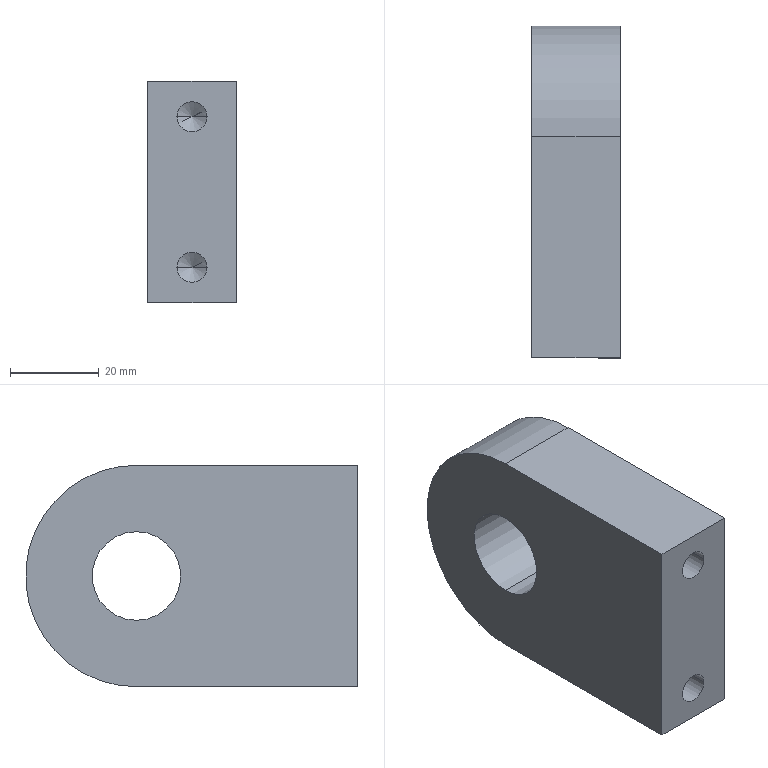Component | SolidWorks | BracketOne-1 | 1 solid | 16 faces | box 20 x 75 x 50 mm | volume 62431 mm3 | cylinder 7 | plane 5 | cone 4 | commonest cylinder face diameters 6.8 x4 20 x2 50 x1
build123d program:
from build123d import *

# Parameters (mm, degrees)
SKETCH1_R             = 10
BOSS_EXTRUDE1_DEPTH   = 20
M8_TAPPED_HOLE1_D     = 6.8
M8_TAPPED_HOLE1_DEPTH = 12
M8_TAPPED_HOLE1_TIP   = 2.043


with BuildPart() as part:
    # Sketch1 → Boss-Extrude1 (new body)
    with BuildSketch(Plane.XY):
        with BuildLine():
            Line((-25, 25), (-25, -25))
            Line((-25, -25), (25, -25))
            Line((25, -25), (25, 25))
            ThreePointArc((25, 25), (0, 50), (-25, 25))
        make_face()
        with Locations((0, 25)):
            Circle(SKETCH1_R, mode=Mode.SUBTRACT)
    extrude(amount=BOSS_EXTRUDE1_DEPTH)

    # M8 Tapped Hole1
    with Locations(Plane(origin=(0, -25, 0), x_dir=(-1, 0, 0), z_dir=(0, -1, 0))):
        with Locations((17, -10), (-17, -10)):
            Hole(M8_TAPPED_HOLE1_D / 2, depth=M8_TAPPED_HOLE1_DEPTH)
            with Locations((0, 0, -(M8_TAPPED_HOLE1_DEPTH + M8_TAPPED_HOLE1_TIP / 2))):  # 118° drill point
                Cone(0, M8_TAPPED_HOLE1_D / 2, M8_TAPPED_HOLE1_TIP, mode=Mode.SUBTRACT)


solid = part.part

# Placed as in the assembly
solid = solid.moved(Location((70.246, 37, 355.671), (0, 90, 0)))
STEP:
#1=COLOUR_RGB('',0.7922,0.8196,0.9333);
#2=FILL_AREA_STYLE_COLOUR('',#1);
#3=FILL_AREA_STYLE('',(#2));
#4=SURFACE_STYLE_FILL_AREA(#3);
#5=SURFACE_SIDE_STYLE('',(#4));
#6=SURFACE_STYLE_USAGE(.BOTH.,#5);
#7=PRESENTATION_STYLE_ASSIGNMENT((#6));
#8=CARTESIAN_POINT('',(3.293,0.9449,14.672));
#9=VERTEX_POINT('',#8);
#10=CARTESIAN_POINT('',(3.025,0.9449,14.672));
#11=VERTEX_POINT('',#10);
#12=CARTESIAN_POINT('',(3.159,0.9449,14.672));
#13=DIRECTION('',(0.,-1.,-0.));
#14=DIRECTION('',(-1.,0.,0.));
#15=AXIS2_PLACEMENT_3D('',#12,#13,#14);
#16=CIRCLE('',#15,0.1339);
#17=EDGE_CURVE('',#9,#11,#16,.T.);
#18=ORIENTED_EDGE('',*,*,#17,.F.);
#19=CARTESIAN_POINT('',(3.293,0.4724,14.672));
#20=VERTEX_POINT('',#19);
#21=CARTESIAN_POINT('',(3.293,0.4724,14.672));
#22=DIRECTION('',(0.,-1.,-0.));
#23=VECTOR('',#22,39.37);
#24=LINE('',#21,#23);
#25=EDGE_CURVE('',#9,#20,#24,.T.);
#26=ORIENTED_EDGE('',*,*,#25,.T.);
#27=CARTESIAN_POINT('',(3.025,0.4724,14.672));
#28=VERTEX_POINT('',#27);
#29=CARTESIAN_POINT('',(3.159,0.4724,14.672));
#30=DIRECTION('',(0.,-1.,-0.));
#31=DIRECTION('',(-1.,0.,0.));
#32=AXIS2_PLACEMENT_3D('',#29,#30,#31);
#33=CIRCLE('',#32,0.1339);
#34=EDGE_CURVE('',#20,#28,#33,.T.);
#35=ORIENTED_EDGE('',*,*,#34,.T.);
#36=CARTESIAN_POINT('',(3.025,0.4724,14.672));
#37=DIRECTION('',(0.,-1.,-0.));
#38=VECTOR('',#37,39.37);
#39=LINE('',#36,#38);
#40=EDGE_CURVE('',#11,#28,#39,.T.);
#41=ORIENTED_EDGE('',*,*,#40,.F.);
#42=EDGE_LOOP('',(#18,#26,#35,#41));
#43=FACE_OUTER_BOUND('',#42,.T.);
#44=CARTESIAN_POINT('',(3.159,0.4724,14.672));
#45=DIRECTION('',(0.,-1.,-0.));
#46=DIRECTION('',(-1.,0.,0.));
#47=AXIS2_PLACEMENT_3D('',#44,#45,#46);
#48=CYLINDRICAL_SURFACE('',#47,0.1339);
#49=ADVANCED_FACE('',(#43),#48,.F.);
#50=CARTESIAN_POINT('',(3.159,1.025,14.672));
#51=VERTEX_POINT('',#50);
#52=CARTESIAN_POINT('',(3.025,0.9449,14.672));
#53=DIRECTION('',(-0.8572,-0.515,0.));
#54=VECTOR('',#53,39.37);
#55=LINE('',#52,#54);
#56=EDGE_CURVE('',#51,#11,#55,.T.);
#57=ORIENTED_EDGE('',*,*,#56,.F.);
#58=CARTESIAN_POINT('',(3.293,0.9449,14.672));
#59=DIRECTION('',(0.8572,-0.515,-0.));
#60=VECTOR('',#59,39.37);
#61=LINE('',#58,#60);
#62=EDGE_CURVE('',#51,#9,#61,.T.);
#63=ORIENTED_EDGE('',*,*,#62,.T.);
#64=ORIENTED_EDGE('',*,*,#17,.T.);
#65=EDGE_LOOP('',(#57,#63,#64));
#66=FACE_OUTER_BOUND('',#65,.T.);
#67=CARTESIAN_POINT('',(3.159,0.9449,14.672));
#68=DIRECTION('',(0.,-1.,-0.));
#69=DIRECTION('',(-1.,0.,0.));
#70=AXIS2_PLACEMENT_3D('',#67,#68,#69);
#71=CONICAL_SURFACE('',#70,0.1339,1.03);
#72=ADVANCED_FACE('',(#66),#71,.F.);
#73=CARTESIAN_POINT('',(3.293,0.9449,13.334));
#74=VERTEX_POINT('',#73);
#75=CARTESIAN_POINT('',(3.025,0.9449,13.334));
#76=VERTEX_POINT('',#75);
#77=CARTESIAN_POINT('',(3.159,0.9449,13.334));
#78=DIRECTION('',(0.,-1.,-0.));
#79=DIRECTION('',(-1.,0.,0.));
#80=AXIS2_PLACEMENT_3D('',#77,#78,#79);
#81=CIRCLE('',#80,0.1339);
#82=EDGE_CURVE('',#74,#76,#81,.T.);
#83=ORIENTED_EDGE('',*,*,#82,.F.);
#84=CARTESIAN_POINT('',(3.293,0.4724,13.334));
#85=VERTEX_POINT('',#84);
#86=CARTESIAN_POINT('',(3.293,0.4724,13.334));
#87=DIRECTION('',(0.,-1.,-0.));
#88=VECTOR('',#87,39.37);
#89=LINE('',#86,#88);
#90=EDGE_CURVE('',#74,#85,#89,.T.);
#91=ORIENTED_EDGE('',*,*,#90,.T.);
#92=CARTESIAN_POINT('',(3.025,0.4724,13.334));
#93=VERTEX_POINT('',#92);
#94=CARTESIAN_POINT('',(3.159,0.4724,13.334));
#95=DIRECTION('',(0.,-1.,-0.));
#96=DIRECTION('',(-1.,0.,0.));
#97=AXIS2_PLACEMENT_3D('',#94,#95,#96);
#98=CIRCLE('',#97,0.1339);
#99=EDGE_CURVE('',#85,#93,#98,.T.);
#100=ORIENTED_EDGE('',*,*,#99,.T.);
#101=CARTESIAN_POINT('',(3.025,0.4724,13.334));
#102=DIRECTION('',(0.,-1.,-0.));
#103=VECTOR('',#102,39.37);
#104=LINE('',#101,#103);
#105=EDGE_CURVE('',#76,#93,#104,.T.);
#106=ORIENTED_EDGE('',*,*,#105,.F.);
#107=EDGE_LOOP('',(#83,#91,#100,#106));
#108=FACE_OUTER_BOUND('',#107,.T.);
#109=CARTESIAN_POINT('',(3.159,0.4724,13.334));
#110=DIRECTION('',(0.,-1.,-0.));
#111=DIRECTION('',(-1.,0.,0.));
#112=AXIS2_PLACEMENT_3D('',#109,#110,#111);
#113=CYLINDRICAL_SURFACE('',#112,0.1339);
#114=ADVANCED_FACE('',(#108),#113,.F.);
#115=CARTESIAN_POINT('',(3.159,1.025,13.334));
#116=VERTEX_POINT('',#115);
#117=CARTESIAN_POINT('',(3.025,0.9449,13.334));
#118=DIRECTION('',(-0.8572,-0.515,0.));
#119=VECTOR('',#118,39.37);
#120=LINE('',#117,#119);
#121=EDGE_CURVE('',#116,#76,#120,.T.);
#122=ORIENTED_EDGE('',*,*,#121,.F.);
#123=CARTESIAN_POINT('',(3.293,0.9449,13.334));
#124=DIRECTION('',(0.8572,-0.515,-0.));
#125=VECTOR('',#124,39.37);
#126=LINE('',#123,#125);
#127=EDGE_CURVE('',#116,#74,#126,.T.);
#128=ORIENTED_EDGE('',*,*,#127,.T.);
#129=ORIENTED_EDGE('',*,*,#82,.T.);
#130=EDGE_LOOP('',(#122,#128,#129));
#131=FACE_OUTER_BOUND('',#130,.T.);
#132=CARTESIAN_POINT('',(3.159,0.9449,13.334));
#133=DIRECTION('',(0.,-1.,-0.));
#134=DIRECTION('',(-1.,0.,0.));
#135=AXIS2_PLACEMENT_3D('',#132,#133,#134);
#136=CONICAL_SURFACE('',#135,0.1339,1.03);
#137=ADVANCED_FACE('',(#131),#136,.F.);
#138=CARTESIAN_POINT('',(3.553,2.441,14.396));
#139=VERTEX_POINT('',#138);
#140=CARTESIAN_POINT('',(3.553,2.441,13.609));
#141=VERTEX_POINT('',#140);
#142=CARTESIAN_POINT('',(3.553,2.441,14.003));
#143=DIRECTION('',(1.,0.,-0.));
#144=DIRECTION('',(-0.,0.,-1.));
#145=AXIS2_PLACEMENT_3D('',#142,#143,#144);
#146=CIRCLE('',#145,0.3937);
#147=EDGE_CURVE('',#139,#141,#146,.T.);
#148=ORIENTED_EDGE('',*,*,#147,.T.);
#149=CARTESIAN_POINT('',(2.766,2.441,13.609));
#150=VERTEX_POINT('',#149);
#151=CARTESIAN_POINT('',(3.553,2.441,13.609));
#152=DIRECTION('',(-1.,-0.,0.));
#153=VECTOR('',#152,39.37);
#154=LINE('',#151,#153);
#155=EDGE_CURVE('',#141,#150,#154,.T.);
#156=ORIENTED_EDGE('',*,*,#155,.T.);
#157=CARTESIAN_POINT('',(2.766,2.441,14.396));
#158=VERTEX_POINT('',#157);
#159=CARTESIAN_POINT('',(2.766,2.441,14.003));
#160=DIRECTION('',(1.,0.,-0.));
#161=DIRECTION('',(-0.,0.,-1.));
#162=AXIS2_PLACEMENT_3D('',#159,#160,#161);
#163=CIRCLE('',#162,0.3937);
#164=EDGE_CURVE('',#158,#150,#163,.T.);
#165=ORIENTED_EDGE('',*,*,#164,.F.);
#166=CARTESIAN_POINT('',(3.553,2.441,14.396));
#167=DIRECTION('',(-1.,-0.,0.));
#168=VECTOR('',#167,39.37);
#169=LINE('',#166,#168);
#170=EDGE_CURVE('',#139,#158,#169,.T.);
#171=ORIENTED_EDGE('',*,*,#170,.F.);
#172=EDGE_LOOP('',(#148,#156,#165,#171));
#173=FACE_OUTER_BOUND('',#172,.T.);
#174=CARTESIAN_POINT('',(3.553,2.441,14.003));
#175=DIRECTION('',(-1.,-0.,0.));
#176=DIRECTION('',(0.,0.,1.));
#177=AXIS2_PLACEMENT_3D('',#174,#175,#176);
#178=CYLINDRICAL_SURFACE('',#177,0.3937);
#179=ADVANCED_FACE('',(#173),#178,.F.);
#180=CARTESIAN_POINT('',(3.553,0.4724,13.019));
#181=VERTEX_POINT('',#180);
#182=CARTESIAN_POINT('',(3.553,2.441,13.019));
#183=VERTEX_POINT('',#182);
#184=CARTESIAN_POINT('',(3.553,2.441,13.019));
#185=DIRECTION('',(-0.,1.,0.));
#186=VECTOR('',#185,39.37);
#187=LINE('',#184,#186);
#188=EDGE_CURVE('',#181,#183,#187,.T.);
#189=ORIENTED_EDGE('',*,*,#188,.T.);
#190=CARTESIAN_POINT('',(3.553,2.441,14.987));
#191=VERTEX_POINT('',#190);
#192=CARTESIAN_POINT('',(3.553,2.441,14.003));
#193=DIRECTION('',(1.,0.,-0.));
#194=DIRECTION('',(-0.,0.,-1.));
#195=AXIS2_PLACEMENT_3D('',#192,#193,#194);
#196=CIRCLE('',#195,0.9843);
#197=EDGE_CURVE('',#183,#191,#196,.T.);
#198=ORIENTED_EDGE('',*,*,#197,.T.);
#199=CARTESIAN_POINT('',(3.553,0.4724,14.987));
#200=VERTEX_POINT('',#199);
#201=CARTESIAN_POINT('',(3.553,2.441,14.987));
#202=DIRECTION('',(0.,-1.,-0.));
#203=VECTOR('',#202,39.37);
#204=LINE('',#201,#203);
#205=EDGE_CURVE('',#191,#200,#204,.T.);
#206=ORIENTED_EDGE('',*,*,#205,.T.);
#207=CARTESIAN_POINT('',(3.553,0.4724,14.987));
#208=DIRECTION('',(-0.,0.,-1.));
#209=VECTOR('',#208,39.37);
#210=LINE('',#207,#209);
#211=EDGE_CURVE('',#200,#181,#210,.T.);
#212=ORIENTED_EDGE('',*,*,#211,.T.);
#213=EDGE_LOOP('',(#189,#198,#206,#212));
#214=FACE_OUTER_BOUND('',#213,.T.);
#215=ORIENTED_EDGE('',*,*,#147,.F.);
#216=CARTESIAN_POINT('',(3.553,2.441,14.003));
#217=DIRECTION('',(1.,0.,-0.));
#218=DIRECTION('',(-0.,0.,-1.));
#219=AXIS2_PLACEMENT_3D('',#216,#217,#218);
#220=CIRCLE('',#219,0.3937);
#221=EDGE_CURVE('',#141,#139,#220,.T.);
#222=ORIENTED_EDGE('',*,*,#221,.F.);
#223=EDGE_LOOP('',(#215,#222));
#224=FACE_BOUND('',#223,.T.);
#225=CARTESIAN_POINT('',(3.553,2.441,14.003));
#226=DIRECTION('',(1.,0.,-0.));
#227=DIRECTION('',(-0.,0.,-1.));
#228=AXIS2_PLACEMENT_3D('',#225,#226,#227);
#229=PLANE('',#228);
#230=ADVANCED_FACE('',(#214,#224),#229,.T.);
#231=CARTESIAN_POINT('',(2.766,0.4724,13.019));
#232=VERTEX_POINT('',#231);
#233=CARTESIAN_POINT('',(2.766,2.441,13.019));
#234=VERTEX_POINT('',#233);
#235=CARTESIAN_POINT('',(2.766,2.441,13.019));
#236=DIRECTION('',(-0.,1.,0.));
#237=VECTOR('',#236,39.37);
#238=LINE('',#235,#237);
#239=EDGE_CURVE('',#232,#234,#238,.T.);
#240=ORIENTED_EDGE('',*,*,#239,.F.);
#241=CARTESIAN_POINT('',(2.766,0.4724,14.987));
#242=VERTEX_POINT('',#241);
#243=CARTESIAN_POINT('',(2.766,0.4724,14.987));
#244=DIRECTION('',(-0.,0.,-1.));
#245=VECTOR('',#244,39.37);
#246=LINE('',#243,#245);
#247=EDGE_CURVE('',#242,#232,#246,.T.);
#248=ORIENTED_EDGE('',*,*,#247,.F.);
#249=CARTESIAN_POINT('',(2.766,2.441,14.987));
#250=VERTEX_POINT('',#249);
#251=CARTESIAN_POINT('',(2.766,2.441,14.987));
#252=DIRECTION('',(0.,-1.,-0.));
#253=VECTOR('',#252,39.37);
#254=LINE('',#251,#253);
#255=EDGE_CURVE('',#250,#242,#254,.T.);
#256=ORIENTED_EDGE('',*,*,#255,.F.);
#257=CARTESIAN_POINT('',(2.766,2.441,14.003));
#258=DIRECTION('',(1.,0.,-0.));
#259=DIRECTION('',(-0.,0.,-1.));
#260=AXIS2_PLACEMENT_3D('',#257,#258,#259);
#261=CIRCLE('',#260,0.9843);
#262=EDGE_CURVE('',#234,#250,#261,.T.);
#263=ORIENTED_EDGE('',*,*,#262,.F.);
#264=EDGE_LOOP('',(#240,#248,#256,#263));
#265=FACE_OUTER_BOUND('',#264,.T.);
#266=ORIENTED_EDGE('',*,*,#164,.T.);
#267=CARTESIAN_POINT('',(2.766,2.441,14.003));
#268=DIRECTION('',(1.,0.,-0.));
#269=DIRECTION('',(-0.,0.,-1.));
#270=AXIS2_PLACEMENT_3D('',#267,#268,#269);
#271=CIRCLE('',#270,0.3937);
#272=EDGE_CURVE('',#150,#158,#271,.T.);
#273=ORIENTED_EDGE('',*,*,#272,.T.);
#274=EDGE_LOOP('',(#266,#273));
#275=FACE_BOUND('',#274,.T.);
#276=CARTESIAN_POINT('',(2.766,2.441,14.003));
#277=DIRECTION('',(1.,0.,-0.));
#278=DIRECTION('',(-0.,0.,-1.));
#279=AXIS2_PLACEMENT_3D('',#276,#277,#278);
#280=PLANE('',#279);
#281=ADVANCED_FACE('',(#265,#275),#280,.F.);
#282=ORIENTED_EDGE('',*,*,#239,.T.);
#283=CARTESIAN_POINT('',(3.553,2.441,13.019));
#284=DIRECTION('',(-1.,-0.,0.));
#285=VECTOR('',#284,39.37);
#286=LINE('',#283,#285);
#287=EDGE_CURVE('',#183,#234,#286,.T.);
#288=ORIENTED_EDGE('',*,*,#287,.F.);
#289=ORIENTED_EDGE('',*,*,#188,.F.);
#290=CARTESIAN_POINT('',(3.553,0.4724,13.019));
#291=DIRECTION('',(-1.,-0.,0.));
#292=VECTOR('',#291,39.37);
#293=LINE('',#290,#292);
#294=EDGE_CURVE('',#181,#232,#293,.T.);
#295=ORIENTED_EDGE('',*,*,#294,.T.);
#296=EDGE_LOOP('',(#282,#288,#289,#295));
#297=FACE_OUTER_BOUND('',#296,.T.);
#298=CARTESIAN_POINT('',(3.553,2.441,13.019));
#299=DIRECTION('',(0.,-0.,1.));
#300=DIRECTION('',(0.,-1.,-0.));
#301=AXIS2_PLACEMENT_3D('',#298,#299,#300);
#302=PLANE('',#301);
#303=ADVANCED_FACE('',(#297),#302,.F.);
#304=ORIENTED_EDGE('',*,*,#262,.T.);
#305=CARTESIAN_POINT('',(3.553,2.441,14.987));
#306=DIRECTION('',(-1.,-0.,0.));
#307=VECTOR('',#306,39.37);
#308=LINE('',#305,#307);
#309=EDGE_CURVE('',#191,#250,#308,.T.);
#310=ORIENTED_EDGE('',*,*,#309,.F.);
#311=ORIENTED_EDGE('',*,*,#197,.F.);
#312=ORIENTED_EDGE('',*,*,#287,.T.);
#313=EDGE_LOOP('',(#304,#310,#311,#312));
#314=FACE_OUTER_BOUND('',#313,.T.);
#315=CARTESIAN_POINT('',(3.553,2.441,14.003));
#316=DIRECTION('',(-1.,-0.,0.));
#317=DIRECTION('',(0.,-0.,1.));
#318=AXIS2_PLACEMENT_3D('',#315,#316,#317);
#319=CYLINDRICAL_SURFACE('',#318,0.9843);
#320=ADVANCED_FACE('',(#314),#319,.T.);
#321=ORIENTED_EDGE('',*,*,#255,.T.);
#322=CARTESIAN_POINT('',(3.553,0.4724,14.987));
#323=DIRECTION('',(-1.,-0.,0.));
#324=VECTOR('',#323,39.37);
#325=LINE('',#322,#324);
#326=EDGE_CURVE('',#200,#242,#325,.T.);
#327=ORIENTED_EDGE('',*,*,#326,.F.);
#328=ORIENTED_EDGE('',*,*,#205,.F.);
#329=ORIENTED_EDGE('',*,*,#309,.T.);
#330=EDGE_LOOP('',(#321,#327,#328,#329));
#331=FACE_OUTER_BOUND('',#330,.T.);
#332=CARTESIAN_POINT('',(3.553,2.441,14.987));
#333=DIRECTION('',(-0.,0.,-1.));
#334=DIRECTION('',(-0.,1.,0.));
#335=AXIS2_PLACEMENT_3D('',#332,#333,#334);
#336=PLANE('',#335);
#337=ADVANCED_FACE('',(#331),#336,.F.);
#338=CARTESIAN_POINT('',(3.159,0.4724,14.672));
#339=DIRECTION('',(0.,-1.,-0.));
#340=DIRECTION('',(-1.,0.,0.));
#341=AXIS2_PLACEMENT_3D('',#338,#339,#340);
#342=CIRCLE('',#341,0.1339);
#343=EDGE_CURVE('',#28,#20,#342,.T.);
#344=ORIENTED_EDGE('',*,*,#343,.F.);
#345=ORIENTED_EDGE('',*,*,#34,.F.);
#346=EDGE_LOOP('',(#344,#345));
#347=FACE_BOUND('',#346,.T.);
#348=CARTESIAN_POINT('',(3.159,0.4724,13.334));
#349=DIRECTION('',(0.,-1.,-0.));
#350=DIRECTION('',(-1.,0.,0.));
#351=AXIS2_PLACEMENT_3D('',#348,#349,#350);
#352=CIRCLE('',#351,0.1339);
#353=EDGE_CURVE('',#93,#85,#352,.T.);
#354=ORIENTED_EDGE('',*,*,#353,.F.);
#355=ORIENTED_EDGE('',*,*,#99,.F.);
#356=EDGE_LOOP('',(#354,#355));
#357=FACE_BOUND('',#356,.T.);
#358=ORIENTED_EDGE('',*,*,#247,.T.);
#359=ORIENTED_EDGE('',*,*,#294,.F.);
#360=ORIENTED_EDGE('',*,*,#211,.F.);
#361=ORIENTED_EDGE('',*,*,#326,.T.);
#362=EDGE_LOOP('',(#358,#359,#360,#361));
#363=FACE_OUTER_BOUND('',#362,.T.);
#364=CARTESIAN_POINT('',(3.553,0.4724,14.987));
#365=DIRECTION('',(-0.,1.,0.));
#366=DIRECTION('',(1.,0.,-0.));
#367=AXIS2_PLACEMENT_3D('',#364,#365,#366);
#368=PLANE('',#367);
#369=ADVANCED_FACE('',(#347,#357,#363),#368,.F.);
#370=ORIENTED_EDGE('',*,*,#155,.F.);
#371=ORIENTED_EDGE('',*,*,#221,.T.);
#372=ORIENTED_EDGE('',*,*,#170,.T.);
#373=ORIENTED_EDGE('',*,*,#272,.F.);
#374=EDGE_LOOP('',(#370,#371,#372,#373));
#375=FACE_OUTER_BOUND('',#374,.T.);
#376=CARTESIAN_POINT('',(3.553,2.441,14.003));
#377=DIRECTION('',(-1.,-0.,0.));
#378=DIRECTION('',(0.,0.,1.));
#379=AXIS2_PLACEMENT_3D('',#376,#377,#378);
#380=CYLINDRICAL_SURFACE('',#379,0.3937);
#381=ADVANCED_FACE('',(#375),#380,.F.);
#382=ORIENTED_EDGE('',*,*,#127,.F.);
#383=ORIENTED_EDGE('',*,*,#121,.T.);
#384=CARTESIAN_POINT('',(3.159,0.9449,13.334));
#385=DIRECTION('',(0.,-1.,-0.));
#386=DIRECTION('',(-1.,0.,0.));
#387=AXIS2_PLACEMENT_3D('',#384,#385,#386);
#388=CIRCLE('',#387,0.1339);
#389=EDGE_CURVE('',#76,#74,#388,.T.);
#390=ORIENTED_EDGE('',*,*,#389,.T.);
#391=EDGE_LOOP('',(#382,#383,#390));
#392=FACE_OUTER_BOUND('',#391,.T.);
#393=CARTESIAN_POINT('',(3.159,0.9449,13.334));
#394=DIRECTION('',(0.,-1.,-0.));
#395=DIRECTION('',(-1.,0.,0.));
#396=AXIS2_PLACEMENT_3D('',#393,#394,#395);
#397=CONICAL_SURFACE('',#396,0.1339,1.03);
#398=ADVANCED_FACE('',(#392),#397,.F.);
#399=ORIENTED_EDGE('',*,*,#90,.F.);
#400=ORIENTED_EDGE('',*,*,#389,.F.);
#401=ORIENTED_EDGE('',*,*,#105,.T.);
#402=ORIENTED_EDGE('',*,*,#353,.T.);
#403=EDGE_LOOP('',(#399,#400,#401,#402));
#404=FACE_OUTER_BOUND('',#403,.T.);
#405=CARTESIAN_POINT('',(3.159,0.4724,13.334));
#406=DIRECTION('',(0.,-1.,-0.));
#407=DIRECTION('',(-1.,0.,0.));
#408=AXIS2_PLACEMENT_3D('',#405,#406,#407);
#409=CYLINDRICAL_SURFACE('',#408,0.1339);
#410=ADVANCED_FACE('',(#404),#409,.F.);
#411=ORIENTED_EDGE('',*,*,#62,.F.);
#412=ORIENTED_EDGE('',*,*,#56,.T.);
#413=CARTESIAN_POINT('',(3.159,0.9449,14.672));
#414=DIRECTION('',(0.,-1.,-0.));
#415=DIRECTION('',(-1.,0.,0.));
#416=AXIS2_PLACEMENT_3D('',#413,#414,#415);
#417=CIRCLE('',#416,0.1339);
#418=EDGE_CURVE('',#11,#9,#417,.T.);
#419=ORIENTED_EDGE('',*,*,#418,.T.);
#420=EDGE_LOOP('',(#411,#412,#419));
#421=FACE_OUTER_BOUND('',#420,.T.);
#422=CARTESIAN_POINT('',(3.159,0.9449,14.672));
#423=DIRECTION('',(0.,-1.,-0.));
#424=DIRECTION('',(-1.,0.,0.));
#425=AXIS2_PLACEMENT_3D('',#422,#423,#424);
#426=CONICAL_SURFACE('',#425,0.1339,1.03);
#427=ADVANCED_FACE('',(#421),#426,.F.);
#428=ORIENTED_EDGE('',*,*,#25,.F.);
#429=ORIENTED_EDGE('',*,*,#418,.F.);
#430=ORIENTED_EDGE('',*,*,#40,.T.);
#431=ORIENTED_EDGE('',*,*,#343,.T.);
#432=EDGE_LOOP('',(#428,#429,#430,#431));
#433=FACE_OUTER_BOUND('',#432,.T.);
#434=CARTESIAN_POINT('',(3.159,0.4724,14.672));
#435=DIRECTION('',(0.,-1.,-0.));
#436=DIRECTION('',(-1.,0.,0.));
#437=AXIS2_PLACEMENT_3D('',#434,#435,#436);
#438=CYLINDRICAL_SURFACE('',#437,0.1339);
#439=ADVANCED_FACE('',(#433),#438,.F.);
#440=CLOSED_SHELL('',(#49,#72,#114,#137,#179,#230,#281,#303,#320,#337,#369,#381,#398,#410,#427,#439));
#441=MANIFOLD_SOLID_BREP('',#440);
#442=STYLED_ITEM('',(#7),#441);
#443=PRESENTATION_LAYER_ASSIGNMENT('','',(#442));
#444=(LENGTH_UNIT()NAMED_UNIT(*)SI_UNIT($,.METRE.));
#445=LENGTH_MEASURE_WITH_UNIT(LENGTH_MEASURE(0.0254),#444);
#446=DIMENSIONAL_EXPONENTS(1.,0.,0.,0.,0.,0.,0.);
#447=(CONVERSION_BASED_UNIT('',#445)LENGTH_UNIT()NAMED_UNIT(#446));
#448=UNCERTAINTY_MEASURE_WITH_UNIT(LENGTH_MEASURE(0.00001),#447,'','');
#449=(NAMED_UNIT(*)PLANE_ANGLE_UNIT()SI_UNIT($,.RADIAN.));
#450=(NAMED_UNIT(*)SI_UNIT($,.STERADIAN.)SOLID_ANGLE_UNIT());
#451=(GEOMETRIC_REPRESENTATION_CONTEXT(3)GLOBAL_UNCERTAINTY_ASSIGNED_CONTEXT((#448))GLOBAL_UNIT_ASSIGNED_CONTEXT((#447,#449,#450))REPRESENTATION_CONTEXT('',''));
#452=MECHANICAL_DESIGN_GEOMETRIC_PRESENTATION_REPRESENTATION('',(#442),#451);
#453=CARTESIAN_POINT('',(0.,0.,0.));
#454=DIRECTION('',(0.,0.,1.));
#455=DIRECTION('',(1.,0.,0.));
#456=AXIS2_PLACEMENT_3D('',#453,#454,#455);
#457=(LENGTH_UNIT()NAMED_UNIT(*)SI_UNIT($,.METRE.));
#458=LENGTH_MEASURE_WITH_UNIT(LENGTH_MEASURE(0.0254),#457);
#459=DIMENSIONAL_EXPONENTS(1.,0.,0.,0.,0.,0.,0.);
#460=(CONVERSION_BASED_UNIT('',#458)LENGTH_UNIT()NAMED_UNIT(#459));
#461=UNCERTAINTY_MEASURE_WITH_UNIT(LENGTH_MEASURE(0.00001),#460,'','');
#462=(NAMED_UNIT(*)PLANE_ANGLE_UNIT()SI_UNIT($,.RADIAN.));
#463=(NAMED_UNIT(*)SI_UNIT($,.STERADIAN.)SOLID_ANGLE_UNIT());
#464=(GEOMETRIC_REPRESENTATION_CONTEXT(3)GLOBAL_UNCERTAINTY_ASSIGNED_CONTEXT((#461))GLOBAL_UNIT_ASSIGNED_CONTEXT((#460,#462,#463))REPRESENTATION_CONTEXT('',''));
#465=ADVANCED_BREP_SHAPE_REPRESENTATION('',(#441,#456),#464);